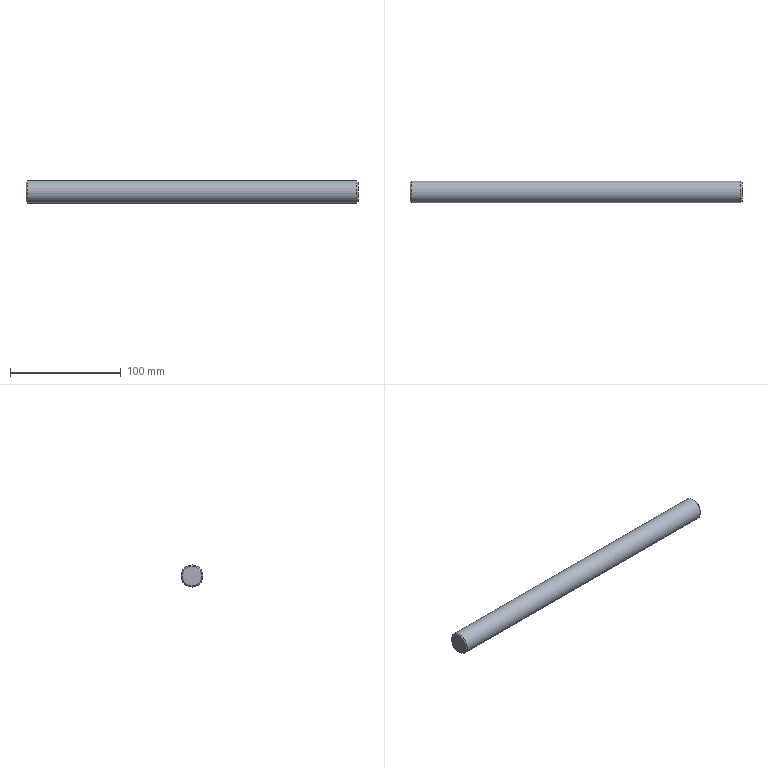Component | NX | LEVER | 1 solid | 5 faces | box 300 x 20 x 20 mm | volume 94187 mm3 | plane 2 | cone 2 | cylinder 1 | commonest cylinder face diameters 20 x1
STEP:
#1=CARTESIAN_POINT('',(0.,0.,0.));
#2=DIRECTION('',(0.,0.,1.));
#3=DIRECTION('',(1.,0.,0.));
#4=AXIS2_PLACEMENT_3D('',#1,#2,#3);
#5=CARTESIAN_POINT('',(150.,-0.,196.));
#6=VERTEX_POINT('',#5);
#7=CARTESIAN_POINT('',(150.,-0.,187.));
#8=DIRECTION('',(1.,0.,0.));
#9=DIRECTION('',(0.,0.,1.));
#10=AXIS2_PLACEMENT_3D('',#7,#8,#9);
#11=CIRCLE('',#10,9.);
#12=CARTESIAN_POINT('',(150.,-0.,187.));
#13=DIRECTION('',(1.,0.,0.));
#14=DIRECTION('',(0.,0.,1.));
#15=AXIS2_PLACEMENT_3D('',#12,#13,#14);
#16=PLANE('',#15);
#17=CARTESIAN_POINT('',(0.,0.));
#18=DIRECTION('',(1.,0.));
#19=AXIS2_PLACEMENT_2D('',#17,#18);
#20=CIRCLE('',#19,9.);
#21=(GEOMETRIC_REPRESENTATION_CONTEXT(2)PARAMETRIC_REPRESENTATION_CONTEXT()REPRESENTATION_CONTEXT('',''));
#22=DEFINITIONAL_REPRESENTATION('',(#20),#21);
#23=PCURVE('',#16,#22);
#24=CARTESIAN_POINT('',(149.,-0.,187.));
#25=DIRECTION('',(-1.,0.,0.));
#26=DIRECTION('',(0.,0.,-1.));
#27=AXIS2_PLACEMENT_3D('',#24,#25,#26);
#28=CONICAL_SURFACE('',#27,10.,0.7854);
#29=CARTESIAN_POINT('',(9.425,-1.));
#30=DIRECTION('',(-1.,0.));
#31=VECTOR('',#30,1.);
#32=LINE('',#29,#31);
#33=(GEOMETRIC_REPRESENTATION_CONTEXT(2)PARAMETRIC_REPRESENTATION_CONTEXT()REPRESENTATION_CONTEXT('',''));
#34=DEFINITIONAL_REPRESENTATION('',(#32),#33);
#35=PCURVE('',#28,#34);
#36=SURFACE_CURVE('',#11,(#23,#35),.PCURVE_S1.);
#37=EDGE_CURVE('',#6,#6,#36,.T.);
#38=ORIENTED_EDGE('',*,*,#37,.T.);
#39=EDGE_LOOP('',(#38));
#40=FACE_BOUND('',#39,.T.);
#41=ADVANCED_FACE('',(#40),#16,.T.);
#42=CARTESIAN_POINT('',(-150.,-0.,178.));
#43=VERTEX_POINT('',#42);
#44=CARTESIAN_POINT('',(-150.,-0.,187.));
#45=DIRECTION('',(-1.,0.,0.));
#46=DIRECTION('',(0.,0.,-1.));
#47=AXIS2_PLACEMENT_3D('',#44,#45,#46);
#48=CIRCLE('',#47,9.);
#49=CARTESIAN_POINT('',(-150.,-0.,187.));
#50=DIRECTION('',(-1.,0.,0.));
#51=DIRECTION('',(0.,0.,-1.));
#52=AXIS2_PLACEMENT_3D('',#49,#50,#51);
#53=PLANE('',#52);
#54=CARTESIAN_POINT('',(0.,0.));
#55=DIRECTION('',(1.,0.));
#56=AXIS2_PLACEMENT_2D('',#54,#55);
#57=CIRCLE('',#56,9.);
#58=(GEOMETRIC_REPRESENTATION_CONTEXT(2)PARAMETRIC_REPRESENTATION_CONTEXT()REPRESENTATION_CONTEXT('',''));
#59=DEFINITIONAL_REPRESENTATION('',(#57),#58);
#60=PCURVE('',#53,#59);
#61=CARTESIAN_POINT('',(-149.,-0.,187.));
#62=DIRECTION('',(1.,0.,0.));
#63=DIRECTION('',(0.,0.,1.));
#64=AXIS2_PLACEMENT_3D('',#61,#62,#63);
#65=CONICAL_SURFACE('',#64,10.,0.7854);
#66=CARTESIAN_POINT('',(9.425,-1.));
#67=DIRECTION('',(-1.,0.));
#68=VECTOR('',#67,1.);
#69=LINE('',#66,#68);
#70=(GEOMETRIC_REPRESENTATION_CONTEXT(2)PARAMETRIC_REPRESENTATION_CONTEXT()REPRESENTATION_CONTEXT('',''));
#71=DEFINITIONAL_REPRESENTATION('',(#69),#70);
#72=PCURVE('',#65,#71);
#73=SURFACE_CURVE('',#48,(#60,#72),.PCURVE_S1.);
#74=EDGE_CURVE('',#43,#43,#73,.T.);
#75=ORIENTED_EDGE('',*,*,#74,.T.);
#76=EDGE_LOOP('',(#75));
#77=FACE_BOUND('',#76,.T.);
#78=ADVANCED_FACE('',(#77),#53,.T.);
#79=CARTESIAN_POINT('',(-149.,-0.,177.));
#80=VERTEX_POINT('',#79);
#81=CARTESIAN_POINT('',(-149.,-0.,197.));
#82=VERTEX_POINT('',#81);
#83=CARTESIAN_POINT('',(-149.,-0.,187.));
#84=DIRECTION('',(1.,0.,0.));
#85=DIRECTION('',(0.,0.,-1.));
#86=AXIS2_PLACEMENT_3D('',#83,#84,#85);
#87=CIRCLE('',#86,10.);
#88=CARTESIAN_POINT('',(-150.,-0.,187.));
#89=DIRECTION('',(1.,0.,0.));
#90=DIRECTION('',(0.,0.,1.));
#91=AXIS2_PLACEMENT_3D('',#88,#89,#90);
#92=CYLINDRICAL_SURFACE('',#91,10.);
#93=CARTESIAN_POINT('',(3.142,1.));
#94=DIRECTION('',(1.,0.));
#95=VECTOR('',#94,1.);
#96=LINE('',#93,#95);
#97=(GEOMETRIC_REPRESENTATION_CONTEXT(2)PARAMETRIC_REPRESENTATION_CONTEXT()REPRESENTATION_CONTEXT('',''));
#98=DEFINITIONAL_REPRESENTATION('',(#96),#97);
#99=PCURVE('',#92,#98);
#100=CARTESIAN_POINT('',(3.142,0.));
#101=DIRECTION('',(1.,0.));
#102=VECTOR('',#101,1.);
#103=LINE('',#100,#102);
#104=(GEOMETRIC_REPRESENTATION_CONTEXT(2)PARAMETRIC_REPRESENTATION_CONTEXT()REPRESENTATION_CONTEXT('',''));
#105=DEFINITIONAL_REPRESENTATION('',(#103),#104);
#106=PCURVE('',#65,#105);
#107=SURFACE_CURVE('',#87,(#99,#106),.PCURVE_S1.);
#108=EDGE_CURVE('',#80,#82,#107,.T.);
#109=ORIENTED_EDGE('',*,*,#108,.T.);
#110=CARTESIAN_POINT('',(149.,-0.,197.));
#111=VERTEX_POINT('',#110);
#112=CARTESIAN_POINT('',(-149.,-0.,197.));
#113=CARTESIAN_POINT('',(149.,-0.,197.));
#114=B_SPLINE_CURVE_WITH_KNOTS('',1,(#112,#113),.UNSPECIFIED.,.F.,.F.,(2,2),(1.,299.),.PIECEWISE_BEZIER_KNOTS.);
#115=CARTESIAN_POINT('',(6.283,0.));
#116=DIRECTION('',(0.,1.));
#117=VECTOR('',#116,1.);
#118=LINE('',#115,#117);
#119=(GEOMETRIC_REPRESENTATION_CONTEXT(2)PARAMETRIC_REPRESENTATION_CONTEXT()REPRESENTATION_CONTEXT('',''));
#120=DEFINITIONAL_REPRESENTATION('',(#118),#119);
#121=PCURVE('',#92,#120);
#122=CARTESIAN_POINT('',(0.,0.));
#123=DIRECTION('',(0.,1.));
#124=VECTOR('',#123,1.);
#125=LINE('',#122,#124);
#126=(GEOMETRIC_REPRESENTATION_CONTEXT(2)PARAMETRIC_REPRESENTATION_CONTEXT()REPRESENTATION_CONTEXT('',''));
#127=DEFINITIONAL_REPRESENTATION('',(#125),#126);
#128=PCURVE('',#92,#127);
#129=SEAM_CURVE('',#114,(#121,#128),.PCURVE_S1.);
#130=EDGE_CURVE('',#82,#111,#129,.T.);
#131=ORIENTED_EDGE('',*,*,#130,.T.);
#132=CARTESIAN_POINT('',(149.,-0.,187.));
#133=DIRECTION('',(-1.,0.,0.));
#134=DIRECTION('',(0.,0.,1.));
#135=AXIS2_PLACEMENT_3D('',#132,#133,#134);
#136=CIRCLE('',#135,10.);
#137=CARTESIAN_POINT('',(6.283,299.));
#138=DIRECTION('',(-1.,0.));
#139=VECTOR('',#138,1.);
#140=LINE('',#137,#139);
#141=(GEOMETRIC_REPRESENTATION_CONTEXT(2)PARAMETRIC_REPRESENTATION_CONTEXT()REPRESENTATION_CONTEXT('',''));
#142=DEFINITIONAL_REPRESENTATION('',(#140),#141);
#143=PCURVE('',#92,#142);
#144=CARTESIAN_POINT('',(3.142,0.));
#145=DIRECTION('',(1.,0.));
#146=VECTOR('',#145,1.);
#147=LINE('',#144,#146);
#148=(GEOMETRIC_REPRESENTATION_CONTEXT(2)PARAMETRIC_REPRESENTATION_CONTEXT()REPRESENTATION_CONTEXT('',''));
#149=DEFINITIONAL_REPRESENTATION('',(#147),#148);
#150=PCURVE('',#28,#149);
#151=SURFACE_CURVE('',#136,(#143,#150),.PCURVE_S1.);
#152=EDGE_CURVE('',#111,#111,#151,.T.);
#153=ORIENTED_EDGE('',*,*,#152,.T.);
#154=ORIENTED_EDGE('',*,*,#130,.F.);
#155=CARTESIAN_POINT('',(-149.,-0.,187.));
#156=DIRECTION('',(1.,0.,0.));
#157=DIRECTION('',(0.,0.,-1.));
#158=AXIS2_PLACEMENT_3D('',#155,#156,#157);
#159=CIRCLE('',#158,10.);
#160=CARTESIAN_POINT('',(-3.142,1.));
#161=DIRECTION('',(1.,0.));
#162=VECTOR('',#161,1.);
#163=LINE('',#160,#162);
#164=(GEOMETRIC_REPRESENTATION_CONTEXT(2)PARAMETRIC_REPRESENTATION_CONTEXT()REPRESENTATION_CONTEXT('',''));
#165=DEFINITIONAL_REPRESENTATION('',(#163),#164);
#166=PCURVE('',#92,#165);
#167=CARTESIAN_POINT('',(3.142,0.));
#168=DIRECTION('',(1.,0.));
#169=VECTOR('',#168,1.);
#170=LINE('',#167,#169);
#171=(GEOMETRIC_REPRESENTATION_CONTEXT(2)PARAMETRIC_REPRESENTATION_CONTEXT()REPRESENTATION_CONTEXT('',''));
#172=DEFINITIONAL_REPRESENTATION('',(#170),#171);
#173=PCURVE('',#65,#172);
#174=SURFACE_CURVE('',#159,(#166,#173),.PCURVE_S1.);
#175=EDGE_CURVE('',#82,#80,#174,.T.);
#176=ORIENTED_EDGE('',*,*,#175,.T.);
#177=EDGE_LOOP('',(#109,#131,#153,#154,#176));
#178=FACE_BOUND('',#177,.T.);
#179=ADVANCED_FACE('',(#178),#92,.T.);
#180=ORIENTED_EDGE('',*,*,#74,.F.);
#181=CARTESIAN_POINT('',(-150.,-0.,178.));
#182=CARTESIAN_POINT('',(-149.,-0.,177.));
#183=B_SPLINE_CURVE_WITH_KNOTS('',1,(#181,#182),.UNSPECIFIED.,.F.,.F.,(2,2),(-1.414,0.),.PIECEWISE_BEZIER_KNOTS.);
#184=CARTESIAN_POINT('',(9.425,0.));
#185=DIRECTION('',(0.,1.));
#186=VECTOR('',#185,1.);
#187=LINE('',#184,#186);
#188=(GEOMETRIC_REPRESENTATION_CONTEXT(2)PARAMETRIC_REPRESENTATION_CONTEXT()REPRESENTATION_CONTEXT('',''));
#189=DEFINITIONAL_REPRESENTATION('',(#187),#188);
#190=PCURVE('',#65,#189);
#191=CARTESIAN_POINT('',(3.142,0.));
#192=DIRECTION('',(0.,1.));
#193=VECTOR('',#192,1.);
#194=LINE('',#191,#193);
#195=(GEOMETRIC_REPRESENTATION_CONTEXT(2)PARAMETRIC_REPRESENTATION_CONTEXT()REPRESENTATION_CONTEXT('',''));
#196=DEFINITIONAL_REPRESENTATION('',(#194),#195);
#197=PCURVE('',#65,#196);
#198=SEAM_CURVE('',#183,(#190,#197),.PCURVE_S1.);
#199=EDGE_CURVE('',#43,#80,#198,.T.);
#200=ORIENTED_EDGE('',*,*,#199,.T.);
#201=ORIENTED_EDGE('',*,*,#175,.F.);
#202=ORIENTED_EDGE('',*,*,#108,.F.);
#203=ORIENTED_EDGE('',*,*,#199,.F.);
#204=EDGE_LOOP('',(#180,#200,#201,#202,#203));
#205=FACE_BOUND('',#204,.T.);
#206=ADVANCED_FACE('',(#205),#65,.T.);
#207=ORIENTED_EDGE('',*,*,#37,.F.);
#208=CARTESIAN_POINT('',(150.,-0.,196.));
#209=CARTESIAN_POINT('',(149.,-0.,197.));
#210=B_SPLINE_CURVE_WITH_KNOTS('',1,(#208,#209),.UNSPECIFIED.,.F.,.F.,(2,2),(-1.414,0.),.PIECEWISE_BEZIER_KNOTS.);
#211=CARTESIAN_POINT('',(9.425,0.));
#212=DIRECTION('',(0.,1.));
#213=VECTOR('',#212,1.);
#214=LINE('',#211,#213);
#215=(GEOMETRIC_REPRESENTATION_CONTEXT(2)PARAMETRIC_REPRESENTATION_CONTEXT()REPRESENTATION_CONTEXT('',''));
#216=DEFINITIONAL_REPRESENTATION('',(#214),#215);
#217=PCURVE('',#28,#216);
#218=CARTESIAN_POINT('',(3.142,0.));
#219=DIRECTION('',(0.,1.));
#220=VECTOR('',#219,1.);
#221=LINE('',#218,#220);
#222=(GEOMETRIC_REPRESENTATION_CONTEXT(2)PARAMETRIC_REPRESENTATION_CONTEXT()REPRESENTATION_CONTEXT('',''));
#223=DEFINITIONAL_REPRESENTATION('',(#221),#222);
#224=PCURVE('',#28,#223);
#225=SEAM_CURVE('',#210,(#217,#224),.PCURVE_S1.);
#226=EDGE_CURVE('',#6,#111,#225,.T.);
#227=ORIENTED_EDGE('',*,*,#226,.T.);
#228=ORIENTED_EDGE('',*,*,#152,.F.);
#229=ORIENTED_EDGE('',*,*,#226,.F.);
#230=EDGE_LOOP('',(#207,#227,#228,#229));
#231=FACE_BOUND('',#230,.T.);
#232=ADVANCED_FACE('',(#231),#28,.T.);
#233=CLOSED_SHELL('',(#41,#78,#179,#206,#232));
#234=MANIFOLD_SOLID_BREP('',#233);
#235=(LENGTH_UNIT()NAMED_UNIT(*)SI_UNIT(.MILLI.,.METRE.));
#236=UNCERTAINTY_MEASURE_WITH_UNIT(LENGTH_MEASURE(0.00001),#235,'','');
#237=(NAMED_UNIT(*)PLANE_ANGLE_UNIT()SI_UNIT($,.RADIAN.));
#238=(NAMED_UNIT(*)SI_UNIT($,.STERADIAN.)SOLID_ANGLE_UNIT());
#239=(GEOMETRIC_REPRESENTATION_CONTEXT(3)GLOBAL_UNCERTAINTY_ASSIGNED_CONTEXT((#236))GLOBAL_UNIT_ASSIGNED_CONTEXT((#235,#237,#238))REPRESENTATION_CONTEXT('',''));
#240=ADVANCED_BREP_SHAPE_REPRESENTATION('',(#4,#234),#239);